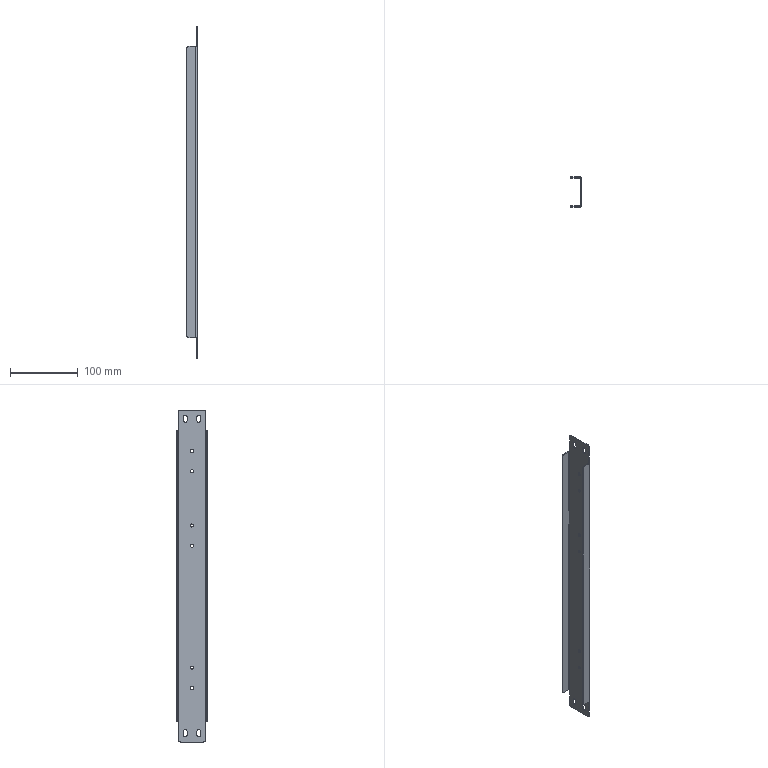Component | SolidWorks | MoldedCaseMountingBeamThree100-2 | 1 solid | 66 faces | volume 48456 mm3 | cylinder 36 | plane 30 | commonest cylinder face diameters 4.5 x12 5.5 x12 6 x8 4.473 x2 1.473 x2